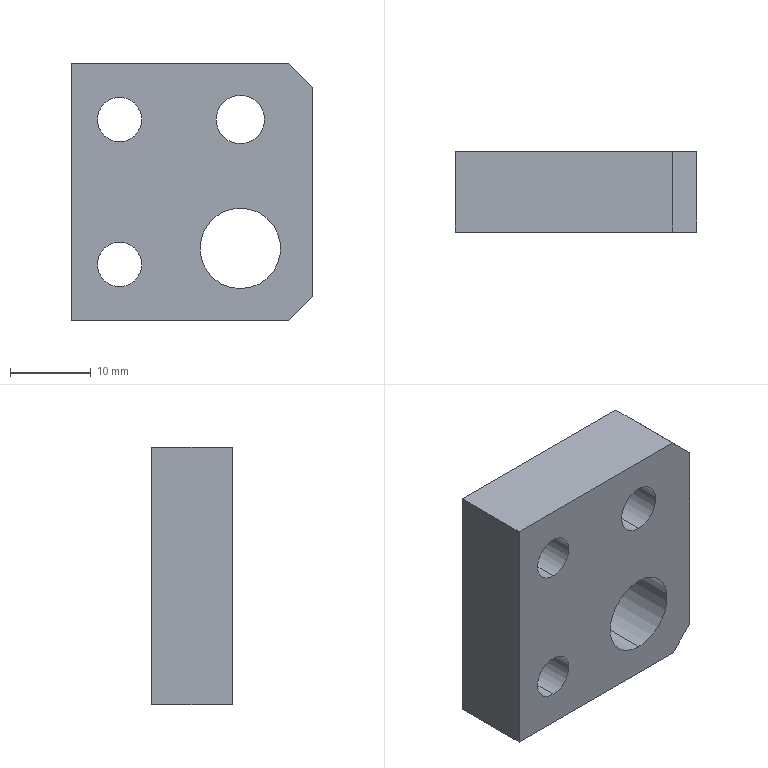Component | SolidWorks | ClampingAssembly-1_A77-3 | 1 solid | 16 faces | box 30 x 10 x 32 mm | volume 7967 mm3 | cylinder 8 | plane 8 | commonest cylinder face diameters 5.5 x4 6 x2 10 x2 | material S45C
build123d program:
from build123d import *

# Parameters (mm, degrees)
SKETCH1_W                  = 32
SKETCH1_H                  = 30
BOSS_EXTRUDE1_DEPTH        = 5
M10X1_0_TAPPED_HOLE1_D     = 10
M6_TAPPED_HOLE1_D          = 6
CHAMFER1_SIZE              = 3
F_5_5_5_5_DIAMETER_HOLE1_D = 5.5


with BuildPart() as part:
    # Sketch1 → Boss-Extrude1 (new, symmetric)
    with BuildSketch(Plane(origin=(0, 0, 0), x_dir=(0, 0, -1), z_dir=(1, 0, 0))):
        Rectangle(SKETCH1_W, SKETCH1_H)
    extrude(amount=BOSS_EXTRUDE1_DEPTH, both=True)

    # M10x1.0 Tapped Hole1 (through all)
    with Locations(Plane(origin=(5, 0, 0), x_dir=(0, 0, -1), z_dir=(1, 0, 0))):
        with Locations((7, 6)):
            Hole(M10X1_0_TAPPED_HOLE1_D / 2)

    # M6 Tapped Hole1 (through all)
    with Locations(Plane(origin=(5, 0, 0), x_dir=(0, 0, -1), z_dir=(1, 0, 0))):
        with Locations((-9, 6)):
            Hole(M6_TAPPED_HOLE1_D / 2)

    # Chamfer1
    chamfer1_edges = [part.edges().sort_by_distance(p)[0] for p in [
        (0, 15, 16),
        (0, 15, -16),
    ]]
    chamfer(chamfer1_edges, length=CHAMFER1_SIZE)

    # 5.5 _5.5_ Diameter Hole1 (through all)
    with Locations(Plane(origin=(5, 0, 0), x_dir=(0, 0, -1), z_dir=(1, 0, 0))):
        with Locations((-9, -9), (9, -9)):
            Hole(F_5_5_5_5_DIAMETER_HOLE1_D / 2)


solid = part.part

# Placed as in the assembly
solid = solid.moved(Location((-14.551, 107.036, 36.5), (0, 0, -90)))
STEP:
#1=CARTESIAN_POINT('',(-0.9272,4.411,1.9));
#2=VERTEX_POINT('',#1);
#3=CARTESIAN_POINT('',(-0.9272,4.411,1.683));
#4=VERTEX_POINT('',#3);
#5=CARTESIAN_POINT('',(-0.9272,4.411,1.791));
#6=DIRECTION('',(0.,-1.,0.));
#7=DIRECTION('',(0.,0.,-1.));
#8=AXIS2_PLACEMENT_3D('',#5,#6,#7);
#9=CIRCLE('',#8,0.1083);
#10=EDGE_CURVE('',#2,#4,#9,.T.);
#11=ORIENTED_EDGE('',*,*,#10,.F.);
#12=CARTESIAN_POINT('',(-0.9272,4.017,1.9));
#13=VERTEX_POINT('',#12);
#14=CARTESIAN_POINT('',(-0.9272,4.017,1.9));
#15=DIRECTION('',(0.,-1.,0.));
#16=VECTOR('',#15,39.37);
#17=LINE('',#14,#16);
#18=EDGE_CURVE('',#2,#13,#17,.T.);
#19=ORIENTED_EDGE('',*,*,#18,.T.);
#20=CARTESIAN_POINT('',(-0.9272,4.017,1.683));
#21=VERTEX_POINT('',#20);
#22=CARTESIAN_POINT('',(-0.9272,4.017,1.791));
#23=DIRECTION('',(0.,-1.,0.));
#24=DIRECTION('',(0.,0.,-1.));
#25=AXIS2_PLACEMENT_3D('',#22,#23,#24);
#26=CIRCLE('',#25,0.1083);
#27=EDGE_CURVE('',#13,#21,#26,.T.);
#28=ORIENTED_EDGE('',*,*,#27,.T.);
#29=CARTESIAN_POINT('',(-0.9272,4.017,1.683));
#30=DIRECTION('',(0.,-1.,0.));
#31=VECTOR('',#30,39.37);
#32=LINE('',#29,#31);
#33=EDGE_CURVE('',#4,#21,#32,.T.);
#34=ORIENTED_EDGE('',*,*,#33,.F.);
#35=EDGE_LOOP('',(#11,#19,#28,#34));
#36=FACE_OUTER_BOUND('',#35,.T.);
#37=CARTESIAN_POINT('',(-0.9272,4.017,1.791));
#38=DIRECTION('',(0.,-1.,0.));
#39=DIRECTION('',(0.,0.,-1.));
#40=AXIS2_PLACEMENT_3D('',#37,#38,#39);
#41=CYLINDRICAL_SURFACE('',#40,0.1083);
#42=ADVANCED_FACE('',(#36),#41,.F.);
#43=CARTESIAN_POINT('',(-0.9272,4.411,1.191));
#44=VERTEX_POINT('',#43);
#45=CARTESIAN_POINT('',(-0.9272,4.411,0.9744));
#46=VERTEX_POINT('',#45);
#47=CARTESIAN_POINT('',(-0.9272,4.411,1.083));
#48=DIRECTION('',(0.,-1.,0.));
#49=DIRECTION('',(0.,0.,-1.));
#50=AXIS2_PLACEMENT_3D('',#47,#48,#49);
#51=CIRCLE('',#50,0.1083);
#52=EDGE_CURVE('',#44,#46,#51,.T.);
#53=ORIENTED_EDGE('',*,*,#52,.F.);
#54=CARTESIAN_POINT('',(-0.9272,4.017,1.191));
#55=VERTEX_POINT('',#54);
#56=CARTESIAN_POINT('',(-0.9272,4.017,1.191));
#57=DIRECTION('',(0.,-1.,0.));
#58=VECTOR('',#57,39.37);
#59=LINE('',#56,#58);
#60=EDGE_CURVE('',#44,#55,#59,.T.);
#61=ORIENTED_EDGE('',*,*,#60,.T.);
#62=CARTESIAN_POINT('',(-0.9272,4.017,0.9744));
#63=VERTEX_POINT('',#62);
#64=CARTESIAN_POINT('',(-0.9272,4.017,1.083));
#65=DIRECTION('',(0.,-1.,0.));
#66=DIRECTION('',(0.,0.,-1.));
#67=AXIS2_PLACEMENT_3D('',#64,#65,#66);
#68=CIRCLE('',#67,0.1083);
#69=EDGE_CURVE('',#55,#63,#68,.T.);
#70=ORIENTED_EDGE('',*,*,#69,.T.);
#71=CARTESIAN_POINT('',(-0.9272,4.017,0.9744));
#72=DIRECTION('',(0.,-1.,0.));
#73=VECTOR('',#72,39.37);
#74=LINE('',#71,#73);
#75=EDGE_CURVE('',#46,#63,#74,.T.);
#76=ORIENTED_EDGE('',*,*,#75,.F.);
#77=EDGE_LOOP('',(#53,#61,#70,#76));
#78=FACE_OUTER_BOUND('',#77,.T.);
#79=CARTESIAN_POINT('',(-0.9272,4.017,1.083));
#80=DIRECTION('',(0.,-1.,0.));
#81=DIRECTION('',(0.,0.,-1.));
#82=AXIS2_PLACEMENT_3D('',#79,#80,#81);
#83=CYLINDRICAL_SURFACE('',#82,0.1083);
#84=ADVANCED_FACE('',(#78),#83,.F.);
#85=CARTESIAN_POINT('',(-0.3366,4.411,1.909));
#86=VERTEX_POINT('',#85);
#87=CARTESIAN_POINT('',(-0.3366,4.411,1.673));
#88=VERTEX_POINT('',#87);
#89=CARTESIAN_POINT('',(-0.3366,4.411,1.791));
#90=DIRECTION('',(0.,-1.,0.));
#91=DIRECTION('',(0.,0.,-1.));
#92=AXIS2_PLACEMENT_3D('',#89,#90,#91);
#93=CIRCLE('',#92,0.1181);
#94=EDGE_CURVE('',#86,#88,#93,.T.);
#95=ORIENTED_EDGE('',*,*,#94,.F.);
#96=CARTESIAN_POINT('',(-0.3366,4.017,1.909));
#97=VERTEX_POINT('',#96);
#98=CARTESIAN_POINT('',(-0.3366,4.017,1.909));
#99=DIRECTION('',(0.,-1.,0.));
#100=VECTOR('',#99,39.37);
#101=LINE('',#98,#100);
#102=EDGE_CURVE('',#86,#97,#101,.T.);
#103=ORIENTED_EDGE('',*,*,#102,.T.);
#104=CARTESIAN_POINT('',(-0.3366,4.017,1.673));
#105=VERTEX_POINT('',#104);
#106=CARTESIAN_POINT('',(-0.3366,4.017,1.791));
#107=DIRECTION('',(0.,-1.,0.));
#108=DIRECTION('',(0.,0.,-1.));
#109=AXIS2_PLACEMENT_3D('',#106,#107,#108);
#110=CIRCLE('',#109,0.1181);
#111=EDGE_CURVE('',#97,#105,#110,.T.);
#112=ORIENTED_EDGE('',*,*,#111,.T.);
#113=CARTESIAN_POINT('',(-0.3366,4.017,1.673));
#114=DIRECTION('',(0.,-1.,0.));
#115=VECTOR('',#114,39.37);
#116=LINE('',#113,#115);
#117=EDGE_CURVE('',#88,#105,#116,.T.);
#118=ORIENTED_EDGE('',*,*,#117,.F.);
#119=EDGE_LOOP('',(#95,#103,#112,#118));
#120=FACE_OUTER_BOUND('',#119,.T.);
#121=CARTESIAN_POINT('',(-0.3366,4.017,1.791));
#122=DIRECTION('',(0.,-1.,0.));
#123=DIRECTION('',(0.,0.,-1.));
#124=AXIS2_PLACEMENT_3D('',#121,#122,#123);
#125=CYLINDRICAL_SURFACE('',#124,0.1181);
#126=ADVANCED_FACE('',(#120),#125,.F.);
#127=CARTESIAN_POINT('',(-0.3366,4.411,1.358));
#128=VERTEX_POINT('',#127);
#129=CARTESIAN_POINT('',(-0.3366,4.411,0.9646));
#130=VERTEX_POINT('',#129);
#131=CARTESIAN_POINT('',(-0.3366,4.411,1.161));
#132=DIRECTION('',(0.,-1.,0.));
#133=DIRECTION('',(0.,0.,-1.));
#134=AXIS2_PLACEMENT_3D('',#131,#132,#133);
#135=CIRCLE('',#134,0.1969);
#136=EDGE_CURVE('',#128,#130,#135,.T.);
#137=ORIENTED_EDGE('',*,*,#136,.F.);
#138=CARTESIAN_POINT('',(-0.3366,4.017,1.358));
#139=VERTEX_POINT('',#138);
#140=CARTESIAN_POINT('',(-0.3366,4.017,1.358));
#141=DIRECTION('',(0.,-1.,0.));
#142=VECTOR('',#141,39.37);
#143=LINE('',#140,#142);
#144=EDGE_CURVE('',#128,#139,#143,.T.);
#145=ORIENTED_EDGE('',*,*,#144,.T.);
#146=CARTESIAN_POINT('',(-0.3366,4.017,0.9646));
#147=VERTEX_POINT('',#146);
#148=CARTESIAN_POINT('',(-0.3366,4.017,1.161));
#149=DIRECTION('',(0.,-1.,0.));
#150=DIRECTION('',(0.,0.,-1.));
#151=AXIS2_PLACEMENT_3D('',#148,#149,#150);
#152=CIRCLE('',#151,0.1969);
#153=EDGE_CURVE('',#139,#147,#152,.T.);
#154=ORIENTED_EDGE('',*,*,#153,.T.);
#155=CARTESIAN_POINT('',(-0.3366,4.017,0.9646));
#156=DIRECTION('',(0.,-1.,0.));
#157=VECTOR('',#156,39.37);
#158=LINE('',#155,#157);
#159=EDGE_CURVE('',#130,#147,#158,.T.);
#160=ORIENTED_EDGE('',*,*,#159,.F.);
#161=EDGE_LOOP('',(#137,#145,#154,#160));
#162=FACE_OUTER_BOUND('',#161,.T.);
#163=CARTESIAN_POINT('',(-0.3366,4.017,1.161));
#164=DIRECTION('',(0.,-1.,0.));
#165=DIRECTION('',(0.,0.,-1.));
#166=AXIS2_PLACEMENT_3D('',#163,#164,#165);
#167=CYLINDRICAL_SURFACE('',#166,0.1969);
#168=ADVANCED_FACE('',(#162),#167,.F.);
#169=CARTESIAN_POINT('',(-1.163,4.411,0.8071));
#170=VERTEX_POINT('',#169);
#171=CARTESIAN_POINT('',(-0.1004,4.411,0.8071));
#172=VERTEX_POINT('',#171);
#173=CARTESIAN_POINT('',(0.01769,4.411,0.8071));
#174=DIRECTION('',(1.,0.,0.));
#175=VECTOR('',#174,39.37);
#176=LINE('',#173,#175);
#177=EDGE_CURVE('',#170,#172,#176,.T.);
#178=ORIENTED_EDGE('',*,*,#177,.T.);
#179=CARTESIAN_POINT('',(-0.1004,4.017,0.8071));
#180=VERTEX_POINT('',#179);
#181=CARTESIAN_POINT('',(-0.1004,4.017,0.8071));
#182=DIRECTION('',(0.,-1.,0.));
#183=VECTOR('',#182,39.37);
#184=LINE('',#181,#183);
#185=EDGE_CURVE('',#172,#180,#184,.T.);
#186=ORIENTED_EDGE('',*,*,#185,.T.);
#187=CARTESIAN_POINT('',(-1.163,4.017,0.8071));
#188=VERTEX_POINT('',#187);
#189=CARTESIAN_POINT('',(0.01769,4.017,0.8071));
#190=DIRECTION('',(1.,0.,0.));
#191=VECTOR('',#190,39.37);
#192=LINE('',#189,#191);
#193=EDGE_CURVE('',#188,#180,#192,.T.);
#194=ORIENTED_EDGE('',*,*,#193,.F.);
#195=CARTESIAN_POINT('',(-1.163,4.017,0.8071));
#196=DIRECTION('',(-0.,1.,-0.));
#197=VECTOR('',#196,39.37);
#198=LINE('',#195,#197);
#199=EDGE_CURVE('',#188,#170,#198,.T.);
#200=ORIENTED_EDGE('',*,*,#199,.T.);
#201=EDGE_LOOP('',(#178,#186,#194,#200));
#202=FACE_OUTER_BOUND('',#201,.T.);
#203=CARTESIAN_POINT('',(0.01769,4.017,0.8071));
#204=DIRECTION('',(-0.,0.,1.));
#205=DIRECTION('',(-1.,-0.,-0.));
#206=AXIS2_PLACEMENT_3D('',#203,#204,#205);
#207=PLANE('',#206);
#208=ADVANCED_FACE('',(#202),#207,.F.);
#209=CARTESIAN_POINT('',(0.01769,4.411,0.9252));
#210=VERTEX_POINT('',#209);
#211=CARTESIAN_POINT('',(0.01769,4.411,1.949));
#212=VERTEX_POINT('',#211);
#213=CARTESIAN_POINT('',(0.01769,4.411,2.067));
#214=DIRECTION('',(-0.,0.,1.));
#215=VECTOR('',#214,39.37);
#216=LINE('',#213,#215);
#217=EDGE_CURVE('',#210,#212,#216,.T.);
#218=ORIENTED_EDGE('',*,*,#217,.T.);
#219=CARTESIAN_POINT('',(0.01769,4.017,1.949));
#220=VERTEX_POINT('',#219);
#221=CARTESIAN_POINT('',(0.01769,4.017,1.949));
#222=DIRECTION('',(0.,-1.,0.));
#223=VECTOR('',#222,39.37);
#224=LINE('',#221,#223);
#225=EDGE_CURVE('',#212,#220,#224,.T.);
#226=ORIENTED_EDGE('',*,*,#225,.T.);
#227=CARTESIAN_POINT('',(0.01769,4.017,0.9252));
#228=VERTEX_POINT('',#227);
#229=CARTESIAN_POINT('',(0.01769,4.017,2.067));
#230=DIRECTION('',(-0.,0.,1.));
#231=VECTOR('',#230,39.37);
#232=LINE('',#229,#231);
#233=EDGE_CURVE('',#228,#220,#232,.T.);
#234=ORIENTED_EDGE('',*,*,#233,.F.);
#235=CARTESIAN_POINT('',(0.01769,4.017,0.9252));
#236=DIRECTION('',(-0.,1.,-0.));
#237=VECTOR('',#236,39.37);
#238=LINE('',#235,#237);
#239=EDGE_CURVE('',#228,#210,#238,.T.);
#240=ORIENTED_EDGE('',*,*,#239,.T.);
#241=EDGE_LOOP('',(#218,#226,#234,#240));
#242=FACE_OUTER_BOUND('',#241,.T.);
#243=CARTESIAN_POINT('',(0.01769,4.017,2.067));
#244=DIRECTION('',(-1.,-0.,-0.));
#245=DIRECTION('',(0.,-0.,-1.));
#246=AXIS2_PLACEMENT_3D('',#243,#244,#245);
#247=PLANE('',#246);
#248=ADVANCED_FACE('',(#242),#247,.F.);
#249=CARTESIAN_POINT('',(-0.1004,4.017,2.067));
#250=VERTEX_POINT('',#249);
#251=CARTESIAN_POINT('',(-1.163,4.017,2.067));
#252=VERTEX_POINT('',#251);
#253=CARTESIAN_POINT('',(0.01769,4.017,2.067));
#254=DIRECTION('',(-1.,-0.,-0.));
#255=VECTOR('',#254,39.37);
#256=LINE('',#253,#255);
#257=EDGE_CURVE('',#250,#252,#256,.T.);
#258=ORIENTED_EDGE('',*,*,#257,.F.);
#259=CARTESIAN_POINT('',(-0.1004,4.411,2.067));
#260=VERTEX_POINT('',#259);
#261=CARTESIAN_POINT('',(-0.1004,4.017,2.067));
#262=DIRECTION('',(-0.,1.,-0.));
#263=VECTOR('',#262,39.37);
#264=LINE('',#261,#263);
#265=EDGE_CURVE('',#250,#260,#264,.T.);
#266=ORIENTED_EDGE('',*,*,#265,.T.);
#267=CARTESIAN_POINT('',(-1.163,4.411,2.067));
#268=VERTEX_POINT('',#267);
#269=CARTESIAN_POINT('',(0.01769,4.411,2.067));
#270=DIRECTION('',(-1.,-0.,-0.));
#271=VECTOR('',#270,39.37);
#272=LINE('',#269,#271);
#273=EDGE_CURVE('',#260,#268,#272,.T.);
#274=ORIENTED_EDGE('',*,*,#273,.T.);
#275=CARTESIAN_POINT('',(-1.163,4.017,2.067));
#276=DIRECTION('',(-0.,1.,-0.));
#277=VECTOR('',#276,39.37);
#278=LINE('',#275,#277);
#279=EDGE_CURVE('',#252,#268,#278,.T.);
#280=ORIENTED_EDGE('',*,*,#279,.F.);
#281=EDGE_LOOP('',(#258,#266,#274,#280));
#282=FACE_OUTER_BOUND('',#281,.T.);
#283=CARTESIAN_POINT('',(0.01769,4.017,2.067));
#284=DIRECTION('',(0.,-0.,-1.));
#285=DIRECTION('',(1.,0.,0.));
#286=AXIS2_PLACEMENT_3D('',#283,#284,#285);
#287=PLANE('',#286);
#288=ADVANCED_FACE('',(#282),#287,.F.);
#289=CARTESIAN_POINT('',(-1.163,4.411,2.067));
#290=DIRECTION('',(0.,-0.,-1.));
#291=VECTOR('',#290,39.37);
#292=LINE('',#289,#291);
#293=EDGE_CURVE('',#268,#170,#292,.T.);
#294=ORIENTED_EDGE('',*,*,#293,.T.);
#295=ORIENTED_EDGE('',*,*,#199,.F.);
#296=CARTESIAN_POINT('',(-1.163,4.017,2.067));
#297=DIRECTION('',(0.,-0.,-1.));
#298=VECTOR('',#297,39.37);
#299=LINE('',#296,#298);
#300=EDGE_CURVE('',#252,#188,#299,.T.);
#301=ORIENTED_EDGE('',*,*,#300,.F.);
#302=ORIENTED_EDGE('',*,*,#279,.T.);
#303=EDGE_LOOP('',(#294,#295,#301,#302));
#304=FACE_OUTER_BOUND('',#303,.T.);
#305=CARTESIAN_POINT('',(-1.163,4.017,2.067));
#306=DIRECTION('',(1.,0.,0.));
#307=DIRECTION('',(-0.,0.,1.));
#308=AXIS2_PLACEMENT_3D('',#305,#306,#307);
#309=PLANE('',#308);
#310=ADVANCED_FACE('',(#304),#309,.F.);
#311=CARTESIAN_POINT('',(-0.9272,4.017,1.791));
#312=DIRECTION('',(0.,-1.,0.));
#313=DIRECTION('',(0.,0.,-1.));
#314=AXIS2_PLACEMENT_3D('',#311,#312,#313);
#315=CIRCLE('',#314,0.1083);
#316=EDGE_CURVE('',#21,#13,#315,.T.);
#317=ORIENTED_EDGE('',*,*,#316,.F.);
#318=ORIENTED_EDGE('',*,*,#27,.F.);
#319=EDGE_LOOP('',(#317,#318));
#320=FACE_BOUND('',#319,.T.);
#321=CARTESIAN_POINT('',(-0.9272,4.017,1.083));
#322=DIRECTION('',(0.,-1.,0.));
#323=DIRECTION('',(0.,0.,-1.));
#324=AXIS2_PLACEMENT_3D('',#321,#322,#323);
#325=CIRCLE('',#324,0.1083);
#326=EDGE_CURVE('',#63,#55,#325,.T.);
#327=ORIENTED_EDGE('',*,*,#326,.F.);
#328=ORIENTED_EDGE('',*,*,#69,.F.);
#329=EDGE_LOOP('',(#327,#328));
#330=FACE_BOUND('',#329,.T.);
#331=CARTESIAN_POINT('',(-0.3366,4.017,1.791));
#332=DIRECTION('',(0.,-1.,0.));
#333=DIRECTION('',(0.,0.,-1.));
#334=AXIS2_PLACEMENT_3D('',#331,#332,#333);
#335=CIRCLE('',#334,0.1181);
#336=EDGE_CURVE('',#105,#97,#335,.T.);
#337=ORIENTED_EDGE('',*,*,#336,.F.);
#338=ORIENTED_EDGE('',*,*,#111,.F.);
#339=EDGE_LOOP('',(#337,#338));
#340=FACE_BOUND('',#339,.T.);
#341=CARTESIAN_POINT('',(-0.3366,4.017,1.161));
#342=DIRECTION('',(0.,-1.,0.));
#343=DIRECTION('',(0.,0.,-1.));
#344=AXIS2_PLACEMENT_3D('',#341,#342,#343);
#345=CIRCLE('',#344,0.1969);
#346=EDGE_CURVE('',#147,#139,#345,.T.);
#347=ORIENTED_EDGE('',*,*,#346,.F.);
#348=ORIENTED_EDGE('',*,*,#153,.F.);
#349=EDGE_LOOP('',(#347,#348));
#350=FACE_BOUND('',#349,.T.);
#351=ORIENTED_EDGE('',*,*,#233,.T.);
#352=CARTESIAN_POINT('',(-0.02168,4.017,1.988));
#353=DIRECTION('',(-0.7071,0.,0.7071));
#354=VECTOR('',#353,39.37);
#355=LINE('',#352,#354);
#356=EDGE_CURVE('',#220,#250,#355,.T.);
#357=ORIENTED_EDGE('',*,*,#356,.T.);
#358=ORIENTED_EDGE('',*,*,#257,.T.);
#359=ORIENTED_EDGE('',*,*,#300,.T.);
#360=ORIENTED_EDGE('',*,*,#193,.T.);
#361=CARTESIAN_POINT('',(-0.02168,4.017,0.8858));
#362=DIRECTION('',(0.7071,0.,0.7071));
#363=VECTOR('',#362,39.37);
#364=LINE('',#361,#363);
#365=EDGE_CURVE('',#180,#228,#364,.T.);
#366=ORIENTED_EDGE('',*,*,#365,.T.);
#367=EDGE_LOOP('',(#351,#357,#358,#359,#360,#366));
#368=FACE_OUTER_BOUND('',#367,.T.);
#369=CARTESIAN_POINT('',(-0.5729,4.017,1.437));
#370=DIRECTION('',(0.,-1.,0.));
#371=DIRECTION('',(0.,-0.,-1.));
#372=AXIS2_PLACEMENT_3D('',#369,#370,#371);
#373=PLANE('',#372);
#374=ADVANCED_FACE('',(#320,#330,#340,#350,#368),#373,.T.);
#375=CARTESIAN_POINT('',(-0.9272,4.411,1.791));
#376=DIRECTION('',(0.,-1.,0.));
#377=DIRECTION('',(0.,0.,-1.));
#378=AXIS2_PLACEMENT_3D('',#375,#376,#377);
#379=CIRCLE('',#378,0.1083);
#380=EDGE_CURVE('',#4,#2,#379,.T.);
#381=ORIENTED_EDGE('',*,*,#380,.T.);
#382=ORIENTED_EDGE('',*,*,#10,.T.);
#383=EDGE_LOOP('',(#381,#382));
#384=FACE_BOUND('',#383,.T.);
#385=CARTESIAN_POINT('',(-0.9272,4.411,1.083));
#386=DIRECTION('',(0.,-1.,0.));
#387=DIRECTION('',(0.,0.,-1.));
#388=AXIS2_PLACEMENT_3D('',#385,#386,#387);
#389=CIRCLE('',#388,0.1083);
#390=EDGE_CURVE('',#46,#44,#389,.T.);
#391=ORIENTED_EDGE('',*,*,#390,.T.);
#392=ORIENTED_EDGE('',*,*,#52,.T.);
#393=EDGE_LOOP('',(#391,#392));
#394=FACE_BOUND('',#393,.T.);
#395=CARTESIAN_POINT('',(-0.3366,4.411,1.791));
#396=DIRECTION('',(0.,-1.,0.));
#397=DIRECTION('',(0.,0.,-1.));
#398=AXIS2_PLACEMENT_3D('',#395,#396,#397);
#399=CIRCLE('',#398,0.1181);
#400=EDGE_CURVE('',#88,#86,#399,.T.);
#401=ORIENTED_EDGE('',*,*,#400,.T.);
#402=ORIENTED_EDGE('',*,*,#94,.T.);
#403=EDGE_LOOP('',(#401,#402));
#404=FACE_BOUND('',#403,.T.);
#405=CARTESIAN_POINT('',(-0.3366,4.411,1.161));
#406=DIRECTION('',(0.,-1.,0.));
#407=DIRECTION('',(0.,0.,-1.));
#408=AXIS2_PLACEMENT_3D('',#405,#406,#407);
#409=CIRCLE('',#408,0.1969);
#410=EDGE_CURVE('',#130,#128,#409,.T.);
#411=ORIENTED_EDGE('',*,*,#410,.T.);
#412=ORIENTED_EDGE('',*,*,#136,.T.);
#413=EDGE_LOOP('',(#411,#412));
#414=FACE_BOUND('',#413,.T.);
#415=ORIENTED_EDGE('',*,*,#273,.F.);
#416=CARTESIAN_POINT('',(-0.1004,4.411,2.067));
#417=DIRECTION('',(0.7071,-0.,-0.7071));
#418=VECTOR('',#417,39.37);
#419=LINE('',#416,#418);
#420=EDGE_CURVE('',#260,#212,#419,.T.);
#421=ORIENTED_EDGE('',*,*,#420,.T.);
#422=ORIENTED_EDGE('',*,*,#217,.F.);
#423=CARTESIAN_POINT('',(0.01769,4.411,0.9252));
#424=DIRECTION('',(-0.7071,-0.,-0.7071));
#425=VECTOR('',#424,39.37);
#426=LINE('',#423,#425);
#427=EDGE_CURVE('',#210,#172,#426,.T.);
#428=ORIENTED_EDGE('',*,*,#427,.T.);
#429=ORIENTED_EDGE('',*,*,#177,.F.);
#430=ORIENTED_EDGE('',*,*,#293,.F.);
#431=EDGE_LOOP('',(#415,#421,#422,#428,#429,#430));
#432=FACE_OUTER_BOUND('',#431,.T.);
#433=CARTESIAN_POINT('',(-0.5729,4.411,1.437));
#434=DIRECTION('',(0.,-1.,0.));
#435=DIRECTION('',(0.,-0.,-1.));
#436=AXIS2_PLACEMENT_3D('',#433,#434,#435);
#437=PLANE('',#436);
#438=ADVANCED_FACE('',(#384,#394,#404,#414,#432),#437,.F.);
#439=ORIENTED_EDGE('',*,*,#144,.F.);
#440=ORIENTED_EDGE('',*,*,#410,.F.);
#441=ORIENTED_EDGE('',*,*,#159,.T.);
#442=ORIENTED_EDGE('',*,*,#346,.T.);
#443=EDGE_LOOP('',(#439,#440,#441,#442));
#444=FACE_OUTER_BOUND('',#443,.T.);
#445=CARTESIAN_POINT('',(-0.3366,4.017,1.161));
#446=DIRECTION('',(0.,-1.,0.));
#447=DIRECTION('',(0.,0.,-1.));
#448=AXIS2_PLACEMENT_3D('',#445,#446,#447);
#449=CYLINDRICAL_SURFACE('',#448,0.1969);
#450=ADVANCED_FACE('',(#444),#449,.F.);
#451=ORIENTED_EDGE('',*,*,#102,.F.);
#452=ORIENTED_EDGE('',*,*,#400,.F.);
#453=ORIENTED_EDGE('',*,*,#117,.T.);
#454=ORIENTED_EDGE('',*,*,#336,.T.);
#455=EDGE_LOOP('',(#451,#452,#453,#454));
#456=FACE_OUTER_BOUND('',#455,.T.);
#457=CARTESIAN_POINT('',(-0.3366,4.017,1.791));
#458=DIRECTION('',(0.,-1.,0.));
#459=DIRECTION('',(0.,0.,-1.));
#460=AXIS2_PLACEMENT_3D('',#457,#458,#459);
#461=CYLINDRICAL_SURFACE('',#460,0.1181);
#462=ADVANCED_FACE('',(#456),#461,.F.);
#463=ORIENTED_EDGE('',*,*,#356,.F.);
#464=ORIENTED_EDGE('',*,*,#225,.F.);
#465=ORIENTED_EDGE('',*,*,#420,.F.);
#466=ORIENTED_EDGE('',*,*,#265,.F.);
#467=EDGE_LOOP('',(#463,#464,#465,#466));
#468=FACE_OUTER_BOUND('',#467,.T.);
#469=CARTESIAN_POINT('',(-0.1004,4.017,2.067));
#470=DIRECTION('',(-0.7071,-0.,-0.7071));
#471=DIRECTION('',(-0.,1.,-0.));
#472=AXIS2_PLACEMENT_3D('',#469,#470,#471);
#473=PLANE('',#472);
#474=ADVANCED_FACE('',(#468),#473,.F.);
#475=ORIENTED_EDGE('',*,*,#365,.F.);
#476=ORIENTED_EDGE('',*,*,#185,.F.);
#477=ORIENTED_EDGE('',*,*,#427,.F.);
#478=ORIENTED_EDGE('',*,*,#239,.F.);
#479=EDGE_LOOP('',(#475,#476,#477,#478));
#480=FACE_OUTER_BOUND('',#479,.T.);
#481=CARTESIAN_POINT('',(0.01769,4.017,0.9252));
#482=DIRECTION('',(-0.7071,0.,0.7071));
#483=DIRECTION('',(-0.,1.,-0.));
#484=AXIS2_PLACEMENT_3D('',#481,#482,#483);
#485=PLANE('',#484);
#486=ADVANCED_FACE('',(#480),#485,.F.);
#487=ORIENTED_EDGE('',*,*,#60,.F.);
#488=ORIENTED_EDGE('',*,*,#390,.F.);
#489=ORIENTED_EDGE('',*,*,#75,.T.);
#490=ORIENTED_EDGE('',*,*,#326,.T.);
#491=EDGE_LOOP('',(#487,#488,#489,#490));
#492=FACE_OUTER_BOUND('',#491,.T.);
#493=CARTESIAN_POINT('',(-0.9272,4.017,1.083));
#494=DIRECTION('',(0.,-1.,0.));
#495=DIRECTION('',(0.,0.,-1.));
#496=AXIS2_PLACEMENT_3D('',#493,#494,#495);
#497=CYLINDRICAL_SURFACE('',#496,0.1083);
#498=ADVANCED_FACE('',(#492),#497,.F.);
#499=ORIENTED_EDGE('',*,*,#18,.F.);
#500=ORIENTED_EDGE('',*,*,#380,.F.);
#501=ORIENTED_EDGE('',*,*,#33,.T.);
#502=ORIENTED_EDGE('',*,*,#316,.T.);
#503=EDGE_LOOP('',(#499,#500,#501,#502));
#504=FACE_OUTER_BOUND('',#503,.T.);
#505=CARTESIAN_POINT('',(-0.9272,4.017,1.791));
#506=DIRECTION('',(0.,-1.,0.));
#507=DIRECTION('',(0.,0.,-1.));
#508=AXIS2_PLACEMENT_3D('',#505,#506,#507);
#509=CYLINDRICAL_SURFACE('',#508,0.1083);
#510=ADVANCED_FACE('',(#504),#509,.F.);
#511=CLOSED_SHELL('',(#42,#84,#126,#168,#208,#248,#288,#310,#374,#438,#450,#462,#474,#486,#498,#510));
#512=MANIFOLD_SOLID_BREP('',#511);
#513=CARTESIAN_POINT('',(0.,0.,0.));
#514=DIRECTION('',(0.,0.,1.));
#515=DIRECTION('',(1.,0.,0.));
#516=AXIS2_PLACEMENT_3D('',#513,#514,#515);
#517=(LENGTH_UNIT()NAMED_UNIT(*)SI_UNIT($,.METRE.));
#518=LENGTH_MEASURE_WITH_UNIT(LENGTH_MEASURE(0.0254),#517);
#519=DIMENSIONAL_EXPONENTS(1.,0.,0.,0.,0.,0.,0.);
#520=(CONVERSION_BASED_UNIT('',#518)LENGTH_UNIT()NAMED_UNIT(#519));
#521=UNCERTAINTY_MEASURE_WITH_UNIT(LENGTH_MEASURE(0.00001),#520,'','');
#522=(NAMED_UNIT(*)PLANE_ANGLE_UNIT()SI_UNIT($,.RADIAN.));
#523=(NAMED_UNIT(*)SI_UNIT($,.STERADIAN.)SOLID_ANGLE_UNIT());
#524=(GEOMETRIC_REPRESENTATION_CONTEXT(3)GLOBAL_UNCERTAINTY_ASSIGNED_CONTEXT((#521))GLOBAL_UNIT_ASSIGNED_CONTEXT((#520,#522,#523))REPRESENTATION_CONTEXT('',''));
#525=ADVANCED_BREP_SHAPE_REPRESENTATION('',(#512,#516),#524);
#526=COLOUR_RGB('',0.7922,0.8196,0.9333);
#527=FILL_AREA_STYLE_COLOUR('',#526);
#528=FILL_AREA_STYLE('',(#527));
#529=SURFACE_STYLE_FILL_AREA(#528);
#530=SURFACE_SIDE_STYLE('',(#529));
#531=SURFACE_STYLE_USAGE(.BOTH.,#530);
#532=PRESENTATION_STYLE_ASSIGNMENT((#531));
#533=STYLED_ITEM('',(#532),#512);
#534=PRESENTATION_LAYER_ASSIGNMENT('','',(#533));
#535=(LENGTH_UNIT()NAMED_UNIT(*)SI_UNIT($,.METRE.));
#536=LENGTH_MEASURE_WITH_UNIT(LENGTH_MEASURE(0.0254),#535);
#537=DIMENSIONAL_EXPONENTS(1.,0.,0.,0.,0.,0.,0.);
#538=(CONVERSION_BASED_UNIT('',#536)LENGTH_UNIT()NAMED_UNIT(#537));
#539=UNCERTAINTY_MEASURE_WITH_UNIT(LENGTH_MEASURE(0.00001),#538,'','');
#540=(NAMED_UNIT(*)PLANE_ANGLE_UNIT()SI_UNIT($,.RADIAN.));
#541=(NAMED_UNIT(*)SI_UNIT($,.STERADIAN.)SOLID_ANGLE_UNIT());
#542=(GEOMETRIC_REPRESENTATION_CONTEXT(3)GLOBAL_UNCERTAINTY_ASSIGNED_CONTEXT((#539))GLOBAL_UNIT_ASSIGNED_CONTEXT((#538,#540,#541))REPRESENTATION_CONTEXT('',''));
#543=MECHANICAL_DESIGN_GEOMETRIC_PRESENTATION_REPRESENTATION('',(#533),#542);